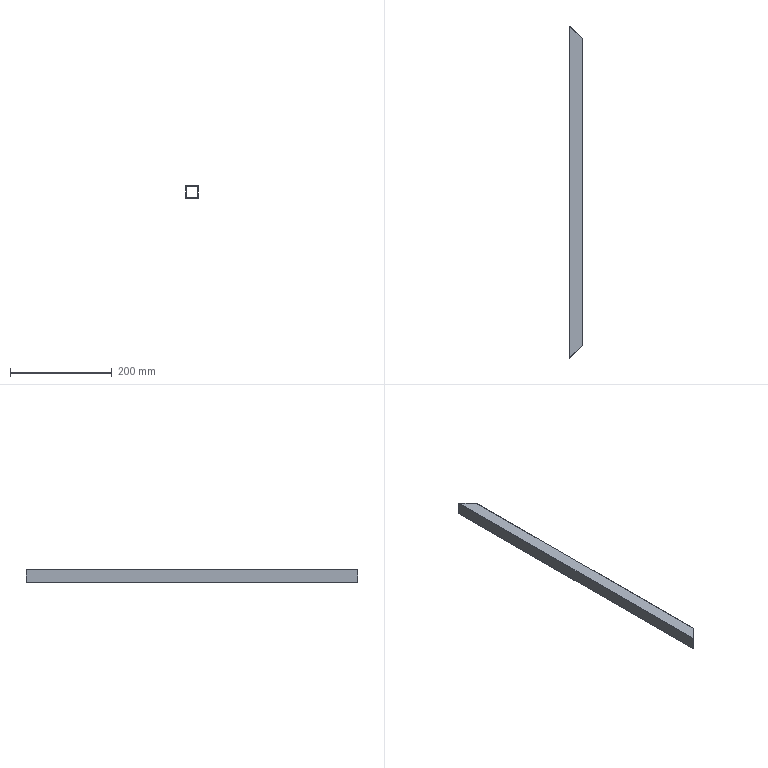Component | SolidWorks | dbj2-1_w7-1 | 1 solid | 10 faces | box 25 x 654 x 25 mm | volume 60384 mm3 | plane 10
build123d program:
from build123d import *

# Parameters (mm, degrees)
SKETCH1_W               = 25
SKETCH1_H               = 25
SKETCH1_W_2             = 23
SKETCH1_H_2             = 23
EXTRUDE_THIN1_DEPTH     = 654
CUT_EXTRUDE1_DEPTH      = 655.597
CUT_EXTRUDE1_DEPTH_BACK = 655.597
CUT_EXTRUDE2_DEPTH      = 655.597
CUT_EXTRUDE2_DEPTH_BACK = 655.597


with BuildPart() as part:
    # Sketch1 → Extrude-Thin1 (new body)
    with BuildSketch(Plane.XY):
        Rectangle(SKETCH1_W, SKETCH1_H)
        Rectangle(SKETCH1_W_2, SKETCH1_H_2, mode=Mode.SUBTRACT)
    extrude(amount=EXTRUDE_THIN1_DEPTH)

    # Sketch2 → Cut-Extrude1 (cut, two sides: drawn at the far end of the back side and taken through both)
    with BuildSketch(Plane(origin=(12.5, 0, 0), x_dir=(0, 0, -1), z_dir=(1, 0, 0)).offset(-CUT_EXTRUDE1_DEPTH_BACK)):
        Polygon((-1586.642, 945.142), (-654, 12.5), (-629, -12.5), (303.642, -945.142), (-1561.642, -2810.427), (-3451.927, -920.142), align=None)
    extrude(amount=CUT_EXTRUDE1_DEPTH + CUT_EXTRUDE1_DEPTH_BACK, mode=Mode.SUBTRACT)

    # Sketch3 → Cut-Extrude2 (cut, two sides: drawn at the far end of the back side and taken through both)
    with BuildSketch(Plane(origin=(12.5, 0, 0), x_dir=(0, 0, -1), z_dir=(1, 0, 0)).offset(-CUT_EXTRUDE2_DEPTH_BACK)):
        Polygon((932.642, 945.142), (0, 12.5), (-25, -12.5), (-957.642, -945.142), (907.642, -2810.427), (2797.927, -920.142), align=None)
    extrude(amount=CUT_EXTRUDE2_DEPTH + CUT_EXTRUDE2_DEPTH_BACK, mode=Mode.SUBTRACT)


solid = part.part

# Placed as in the assembly
solid = solid.moved(Location((-215.5, 726.75, -13.5), (90, 0, 90)))
STEP:
#1=CARTESIAN_POINT('',(-7.992,27.628,-1.024));
#2=VERTEX_POINT('',#1);
#3=CARTESIAN_POINT('',(-8.976,28.612,-1.024));
#4=VERTEX_POINT('',#3);
#5=CARTESIAN_POINT('',(4.39,15.246,-1.024));
#6=DIRECTION('',(-0.7071,0.7071,-0.));
#7=VECTOR('',#6,39.37);
#8=LINE('',#5,#7);
#9=EDGE_CURVE('',#2,#4,#8,.T.);
#10=ORIENTED_EDGE('',*,*,#9,.F.);
#11=CARTESIAN_POINT('',(-7.992,3.848,-1.024));
#12=VERTEX_POINT('',#11);
#13=CARTESIAN_POINT('',(-7.992,2.864,-1.024));
#14=DIRECTION('',(-0.,1.,-0.));
#15=VECTOR('',#14,39.37);
#16=LINE('',#13,#15);
#17=EDGE_CURVE('',#12,#2,#16,.T.);
#18=ORIENTED_EDGE('',*,*,#17,.F.);
#19=CARTESIAN_POINT('',(-8.976,2.864,-1.024));
#20=VERTEX_POINT('',#19);
#21=CARTESIAN_POINT('',(-8.484,3.356,-1.024));
#22=DIRECTION('',(-0.7071,-0.7071,-0.));
#23=VECTOR('',#22,39.37);
#24=LINE('',#21,#23);
#25=EDGE_CURVE('',#12,#20,#24,.T.);
#26=ORIENTED_EDGE('',*,*,#25,.T.);
#27=CARTESIAN_POINT('',(-8.976,2.864,-1.024));
#28=DIRECTION('',(-0.,1.,-0.));
#29=VECTOR('',#28,39.37);
#30=LINE('',#27,#29);
#31=EDGE_CURVE('',#20,#4,#30,.T.);
#32=ORIENTED_EDGE('',*,*,#31,.T.);
#33=EDGE_LOOP('',(#10,#18,#26,#32));
#34=FACE_OUTER_BOUND('',#33,.T.);
#35=CARTESIAN_POINT('',(-7.992,2.864,-1.024));
#36=DIRECTION('',(-0.,0.,1.));
#37=DIRECTION('',(-0.,1.,-0.));
#38=AXIS2_PLACEMENT_3D('',#35,#36,#37);
#39=PLANE('',#38);
#40=ADVANCED_FACE('',(#34),#39,.F.);
#41=CARTESIAN_POINT('',(-7.992,27.628,-0.03937));
#42=VERTEX_POINT('',#41);
#43=CARTESIAN_POINT('',(-7.992,27.628,33.423));
#44=DIRECTION('',(0.,0.,-1.));
#45=VECTOR('',#44,39.37);
#46=LINE('',#43,#45);
#47=EDGE_CURVE('',#42,#2,#46,.T.);
#48=ORIENTED_EDGE('',*,*,#47,.F.);
#49=CARTESIAN_POINT('',(-7.992,3.848,-0.03937));
#50=VERTEX_POINT('',#49);
#51=CARTESIAN_POINT('',(-7.992,2.864,-0.03937));
#52=DIRECTION('',(-0.,1.,-0.));
#53=VECTOR('',#52,39.37);
#54=LINE('',#51,#53);
#55=EDGE_CURVE('',#50,#42,#54,.T.);
#56=ORIENTED_EDGE('',*,*,#55,.F.);
#57=CARTESIAN_POINT('',(-7.992,3.848,33.423));
#58=DIRECTION('',(0.,0.,-1.));
#59=VECTOR('',#58,39.37);
#60=LINE('',#57,#59);
#61=EDGE_CURVE('',#50,#12,#60,.T.);
#62=ORIENTED_EDGE('',*,*,#61,.T.);
#63=ORIENTED_EDGE('',*,*,#17,.T.);
#64=EDGE_LOOP('',(#48,#56,#62,#63));
#65=FACE_OUTER_BOUND('',#64,.T.);
#66=CARTESIAN_POINT('',(-7.992,2.864,-0.03937));
#67=DIRECTION('',(-1.,-0.,-0.));
#68=DIRECTION('',(0.,-1.,0.));
#69=AXIS2_PLACEMENT_3D('',#66,#67,#68);
#70=PLANE('',#69);
#71=ADVANCED_FACE('',(#65),#70,.F.);
#72=CARTESIAN_POINT('',(-8.976,28.612,-0.03937));
#73=VERTEX_POINT('',#72);
#74=CARTESIAN_POINT('',(4.39,15.246,-0.03937));
#75=DIRECTION('',(0.7071,-0.7071,0.));
#76=VECTOR('',#75,39.37);
#77=LINE('',#74,#76);
#78=EDGE_CURVE('',#73,#42,#77,.T.);
#79=ORIENTED_EDGE('',*,*,#78,.F.);
#80=CARTESIAN_POINT('',(-8.976,2.864,-0.03937));
#81=VERTEX_POINT('',#80);
#82=CARTESIAN_POINT('',(-8.976,2.864,-0.03937));
#83=DIRECTION('',(-0.,1.,-0.));
#84=VECTOR('',#83,39.37);
#85=LINE('',#82,#84);
#86=EDGE_CURVE('',#81,#73,#85,.T.);
#87=ORIENTED_EDGE('',*,*,#86,.F.);
#88=CARTESIAN_POINT('',(-8.484,3.356,-0.03937));
#89=DIRECTION('',(0.7071,0.7071,0.));
#90=VECTOR('',#89,39.37);
#91=LINE('',#88,#90);
#92=EDGE_CURVE('',#81,#50,#91,.T.);
#93=ORIENTED_EDGE('',*,*,#92,.T.);
#94=ORIENTED_EDGE('',*,*,#55,.T.);
#95=EDGE_LOOP('',(#79,#87,#93,#94));
#96=FACE_OUTER_BOUND('',#95,.T.);
#97=CARTESIAN_POINT('',(-7.992,2.864,-0.03937));
#98=DIRECTION('',(0.,-0.,-1.));
#99=DIRECTION('',(0.,-1.,0.));
#100=AXIS2_PLACEMENT_3D('',#97,#98,#99);
#101=PLANE('',#100);
#102=ADVANCED_FACE('',(#96),#101,.F.);
#103=CARTESIAN_POINT('',(-8.031,3.809,-0.9843));
#104=VERTEX_POINT('',#103);
#105=CARTESIAN_POINT('',(-8.031,27.667,-0.9843));
#106=VERTEX_POINT('',#105);
#107=CARTESIAN_POINT('',(-8.031,2.864,-0.9843));
#108=DIRECTION('',(-0.,1.,-0.));
#109=VECTOR('',#108,39.37);
#110=LINE('',#107,#109);
#111=EDGE_CURVE('',#104,#106,#110,.T.);
#112=ORIENTED_EDGE('',*,*,#111,.T.);
#113=CARTESIAN_POINT('',(-8.937,28.573,-0.9843));
#114=VERTEX_POINT('',#113);
#115=CARTESIAN_POINT('',(4.39,15.246,-0.9843));
#116=DIRECTION('',(-0.7071,0.7071,-0.));
#117=VECTOR('',#116,39.37);
#118=LINE('',#115,#117);
#119=EDGE_CURVE('',#106,#114,#118,.T.);
#120=ORIENTED_EDGE('',*,*,#119,.T.);
#121=CARTESIAN_POINT('',(-8.937,2.904,-0.9843));
#122=VERTEX_POINT('',#121);
#123=CARTESIAN_POINT('',(-8.937,2.864,-0.9843));
#124=DIRECTION('',(-0.,1.,-0.));
#125=VECTOR('',#124,39.37);
#126=LINE('',#123,#125);
#127=EDGE_CURVE('',#122,#114,#126,.T.);
#128=ORIENTED_EDGE('',*,*,#127,.F.);
#129=CARTESIAN_POINT('',(-8.484,3.356,-0.9843));
#130=DIRECTION('',(-0.7071,-0.7071,-0.));
#131=VECTOR('',#130,39.37);
#132=LINE('',#129,#131);
#133=EDGE_CURVE('',#104,#122,#132,.T.);
#134=ORIENTED_EDGE('',*,*,#133,.F.);
#135=EDGE_LOOP('',(#112,#120,#128,#134));
#136=FACE_OUTER_BOUND('',#135,.T.);
#137=CARTESIAN_POINT('',(-7.992,2.864,-0.9843));
#138=DIRECTION('',(-0.,0.,1.));
#139=DIRECTION('',(-0.,1.,-0.));
#140=AXIS2_PLACEMENT_3D('',#137,#138,#139);
#141=PLANE('',#140);
#142=ADVANCED_FACE('',(#136),#141,.T.);
#143=CARTESIAN_POINT('',(-8.031,3.809,-0.07874));
#144=VERTEX_POINT('',#143);
#145=CARTESIAN_POINT('',(-8.031,27.667,-0.07874));
#146=VERTEX_POINT('',#145);
#147=CARTESIAN_POINT('',(-8.031,2.864,-0.07874));
#148=DIRECTION('',(-0.,1.,-0.));
#149=VECTOR('',#148,39.37);
#150=LINE('',#147,#149);
#151=EDGE_CURVE('',#144,#146,#150,.T.);
#152=ORIENTED_EDGE('',*,*,#151,.T.);
#153=CARTESIAN_POINT('',(-8.031,27.667,-0.03937));
#154=DIRECTION('',(0.,0.,-1.));
#155=VECTOR('',#154,39.37);
#156=LINE('',#153,#155);
#157=EDGE_CURVE('',#146,#106,#156,.T.);
#158=ORIENTED_EDGE('',*,*,#157,.T.);
#159=ORIENTED_EDGE('',*,*,#111,.F.);
#160=CARTESIAN_POINT('',(-8.031,3.809,-0.03937));
#161=DIRECTION('',(0.,0.,-1.));
#162=VECTOR('',#161,39.37);
#163=LINE('',#160,#162);
#164=EDGE_CURVE('',#144,#104,#163,.T.);
#165=ORIENTED_EDGE('',*,*,#164,.F.);
#166=EDGE_LOOP('',(#152,#158,#159,#165));
#167=FACE_OUTER_BOUND('',#166,.T.);
#168=CARTESIAN_POINT('',(-8.031,2.864,-0.03937));
#169=DIRECTION('',(-1.,-0.,-0.));
#170=DIRECTION('',(0.,-1.,0.));
#171=AXIS2_PLACEMENT_3D('',#168,#169,#170);
#172=PLANE('',#171);
#173=ADVANCED_FACE('',(#167),#172,.T.);
#174=CARTESIAN_POINT('',(-8.937,2.904,-0.07874));
#175=VERTEX_POINT('',#174);
#176=CARTESIAN_POINT('',(-8.937,28.573,-0.07874));
#177=VERTEX_POINT('',#176);
#178=CARTESIAN_POINT('',(-8.937,2.864,-0.07874));
#179=DIRECTION('',(-0.,1.,-0.));
#180=VECTOR('',#179,39.37);
#181=LINE('',#178,#180);
#182=EDGE_CURVE('',#175,#177,#181,.T.);
#183=ORIENTED_EDGE('',*,*,#182,.T.);
#184=CARTESIAN_POINT('',(4.39,15.246,-0.07874));
#185=DIRECTION('',(0.7071,-0.7071,0.));
#186=VECTOR('',#185,39.37);
#187=LINE('',#184,#186);
#188=EDGE_CURVE('',#177,#146,#187,.T.);
#189=ORIENTED_EDGE('',*,*,#188,.T.);
#190=ORIENTED_EDGE('',*,*,#151,.F.);
#191=CARTESIAN_POINT('',(-8.484,3.356,-0.07874));
#192=DIRECTION('',(0.7071,0.7071,0.));
#193=VECTOR('',#192,39.37);
#194=LINE('',#191,#193);
#195=EDGE_CURVE('',#175,#144,#194,.T.);
#196=ORIENTED_EDGE('',*,*,#195,.F.);
#197=EDGE_LOOP('',(#183,#189,#190,#196));
#198=FACE_OUTER_BOUND('',#197,.T.);
#199=CARTESIAN_POINT('',(-7.992,2.864,-0.07874));
#200=DIRECTION('',(0.,-0.,-1.));
#201=DIRECTION('',(0.,-1.,0.));
#202=AXIS2_PLACEMENT_3D('',#199,#200,#201);
#203=PLANE('',#202);
#204=ADVANCED_FACE('',(#198),#203,.T.);
#205=ORIENTED_EDGE('',*,*,#127,.T.);
#206=CARTESIAN_POINT('',(-8.937,28.573,-0.03937));
#207=DIRECTION('',(-0.,0.,1.));
#208=VECTOR('',#207,39.37);
#209=LINE('',#206,#208);
#210=EDGE_CURVE('',#114,#177,#209,.T.);
#211=ORIENTED_EDGE('',*,*,#210,.T.);
#212=ORIENTED_EDGE('',*,*,#182,.F.);
#213=CARTESIAN_POINT('',(-8.937,2.904,-0.03937));
#214=DIRECTION('',(-0.,-0.,1.));
#215=VECTOR('',#214,39.37);
#216=LINE('',#213,#215);
#217=EDGE_CURVE('',#122,#175,#216,.T.);
#218=ORIENTED_EDGE('',*,*,#217,.F.);
#219=EDGE_LOOP('',(#205,#211,#212,#218));
#220=FACE_OUTER_BOUND('',#219,.T.);
#221=CARTESIAN_POINT('',(-8.937,2.864,-0.03937));
#222=DIRECTION('',(1.,0.,0.));
#223=DIRECTION('',(-0.,-0.,1.));
#224=AXIS2_PLACEMENT_3D('',#221,#222,#223);
#225=PLANE('',#224);
#226=ADVANCED_FACE('',(#220),#225,.T.);
#227=CARTESIAN_POINT('',(-8.976,28.612,-0.03937));
#228=DIRECTION('',(0.,0.,-1.));
#229=VECTOR('',#228,39.37);
#230=LINE('',#227,#229);
#231=EDGE_CURVE('',#73,#4,#230,.T.);
#232=ORIENTED_EDGE('',*,*,#231,.T.);
#233=ORIENTED_EDGE('',*,*,#31,.F.);
#234=CARTESIAN_POINT('',(-8.976,2.864,-0.03937));
#235=DIRECTION('',(0.,0.,-1.));
#236=VECTOR('',#235,39.37);
#237=LINE('',#234,#236);
#238=EDGE_CURVE('',#81,#20,#237,.T.);
#239=ORIENTED_EDGE('',*,*,#238,.F.);
#240=ORIENTED_EDGE('',*,*,#86,.T.);
#241=EDGE_LOOP('',(#232,#233,#239,#240));
#242=FACE_OUTER_BOUND('',#241,.T.);
#243=CARTESIAN_POINT('',(-8.976,2.864,-0.03937));
#244=DIRECTION('',(1.,0.,0.));
#245=DIRECTION('',(-0.,-0.,1.));
#246=AXIS2_PLACEMENT_3D('',#243,#244,#245);
#247=PLANE('',#246);
#248=ADVANCED_FACE('',(#242),#247,.F.);
#249=ORIENTED_EDGE('',*,*,#164,.T.);
#250=ORIENTED_EDGE('',*,*,#133,.T.);
#251=ORIENTED_EDGE('',*,*,#217,.T.);
#252=ORIENTED_EDGE('',*,*,#195,.T.);
#253=EDGE_LOOP('',(#249,#250,#251,#252));
#254=FACE_BOUND('',#253,.T.);
#255=ORIENTED_EDGE('',*,*,#25,.F.);
#256=ORIENTED_EDGE('',*,*,#61,.F.);
#257=ORIENTED_EDGE('',*,*,#92,.F.);
#258=ORIENTED_EDGE('',*,*,#238,.T.);
#259=EDGE_LOOP('',(#255,#256,#257,#258));
#260=FACE_OUTER_BOUND('',#259,.T.);
#261=CARTESIAN_POINT('',(-8.976,2.864,33.423));
#262=DIRECTION('',(-0.7071,0.7071,-0.));
#263=DIRECTION('',(-0.7071,-0.7071,-0.));
#264=AXIS2_PLACEMENT_3D('',#261,#262,#263);
#265=PLANE('',#264);
#266=ADVANCED_FACE('',(#254,#260),#265,.F.);
#267=ORIENTED_EDGE('',*,*,#119,.F.);
#268=ORIENTED_EDGE('',*,*,#157,.F.);
#269=ORIENTED_EDGE('',*,*,#188,.F.);
#270=ORIENTED_EDGE('',*,*,#210,.F.);
#271=EDGE_LOOP('',(#267,#268,#269,#270));
#272=FACE_BOUND('',#271,.T.);
#273=ORIENTED_EDGE('',*,*,#47,.T.);
#274=ORIENTED_EDGE('',*,*,#9,.T.);
#275=ORIENTED_EDGE('',*,*,#231,.F.);
#276=ORIENTED_EDGE('',*,*,#78,.T.);
#277=EDGE_LOOP('',(#273,#274,#275,#276));
#278=FACE_OUTER_BOUND('',#277,.T.);
#279=CARTESIAN_POINT('',(-8.976,28.612,33.423));
#280=DIRECTION('',(0.7071,0.7071,0.));
#281=DIRECTION('',(-0.7071,0.7071,-0.));
#282=AXIS2_PLACEMENT_3D('',#279,#280,#281);
#283=PLANE('',#282);
#284=ADVANCED_FACE('',(#272,#278),#283,.T.);
#285=CLOSED_SHELL('',(#40,#71,#102,#142,#173,#204,#226,#248,#266,#284));
#286=MANIFOLD_SOLID_BREP('',#285);
#287=CARTESIAN_POINT('',(0.,0.,0.));
#288=DIRECTION('',(0.,0.,1.));
#289=DIRECTION('',(1.,0.,0.));
#290=AXIS2_PLACEMENT_3D('',#287,#288,#289);
#291=(LENGTH_UNIT()NAMED_UNIT(*)SI_UNIT($,.METRE.));
#292=LENGTH_MEASURE_WITH_UNIT(LENGTH_MEASURE(0.0254),#291);
#293=DIMENSIONAL_EXPONENTS(1.,0.,0.,0.,0.,0.,0.);
#294=(CONVERSION_BASED_UNIT('',#292)LENGTH_UNIT()NAMED_UNIT(#293));
#295=UNCERTAINTY_MEASURE_WITH_UNIT(LENGTH_MEASURE(0.00001),#294,'','');
#296=(NAMED_UNIT(*)PLANE_ANGLE_UNIT()SI_UNIT($,.RADIAN.));
#297=(NAMED_UNIT(*)SI_UNIT($,.STERADIAN.)SOLID_ANGLE_UNIT());
#298=(GEOMETRIC_REPRESENTATION_CONTEXT(3)GLOBAL_UNCERTAINTY_ASSIGNED_CONTEXT((#295))GLOBAL_UNIT_ASSIGNED_CONTEXT((#294,#296,#297))REPRESENTATION_CONTEXT('',''));
#299=ADVANCED_BREP_SHAPE_REPRESENTATION('',(#286,#290),#298);
#300=COLOUR_RGB('',0.7922,0.8196,0.9333);
#301=FILL_AREA_STYLE_COLOUR('',#300);
#302=FILL_AREA_STYLE('',(#301));
#303=SURFACE_STYLE_FILL_AREA(#302);
#304=SURFACE_SIDE_STYLE('',(#303));
#305=SURFACE_STYLE_USAGE(.BOTH.,#304);
#306=PRESENTATION_STYLE_ASSIGNMENT((#305));
#307=STYLED_ITEM('',(#306),#286);
#308=PRESENTATION_LAYER_ASSIGNMENT('','',(#307));
#309=(LENGTH_UNIT()NAMED_UNIT(*)SI_UNIT($,.METRE.));
#310=LENGTH_MEASURE_WITH_UNIT(LENGTH_MEASURE(0.0254),#309);
#311=DIMENSIONAL_EXPONENTS(1.,0.,0.,0.,0.,0.,0.);
#312=(CONVERSION_BASED_UNIT('',#310)LENGTH_UNIT()NAMED_UNIT(#311));
#313=UNCERTAINTY_MEASURE_WITH_UNIT(LENGTH_MEASURE(0.00001),#312,'','');
#314=(NAMED_UNIT(*)PLANE_ANGLE_UNIT()SI_UNIT($,.RADIAN.));
#315=(NAMED_UNIT(*)SI_UNIT($,.STERADIAN.)SOLID_ANGLE_UNIT());
#316=(GEOMETRIC_REPRESENTATION_CONTEXT(3)GLOBAL_UNCERTAINTY_ASSIGNED_CONTEXT((#313))GLOBAL_UNIT_ASSIGNED_CONTEXT((#312,#314,#315))REPRESENTATION_CONTEXT('',''));
#317=MECHANICAL_DESIGN_GEOMETRIC_PRESENTATION_REPRESENTATION('',(#307),#316);